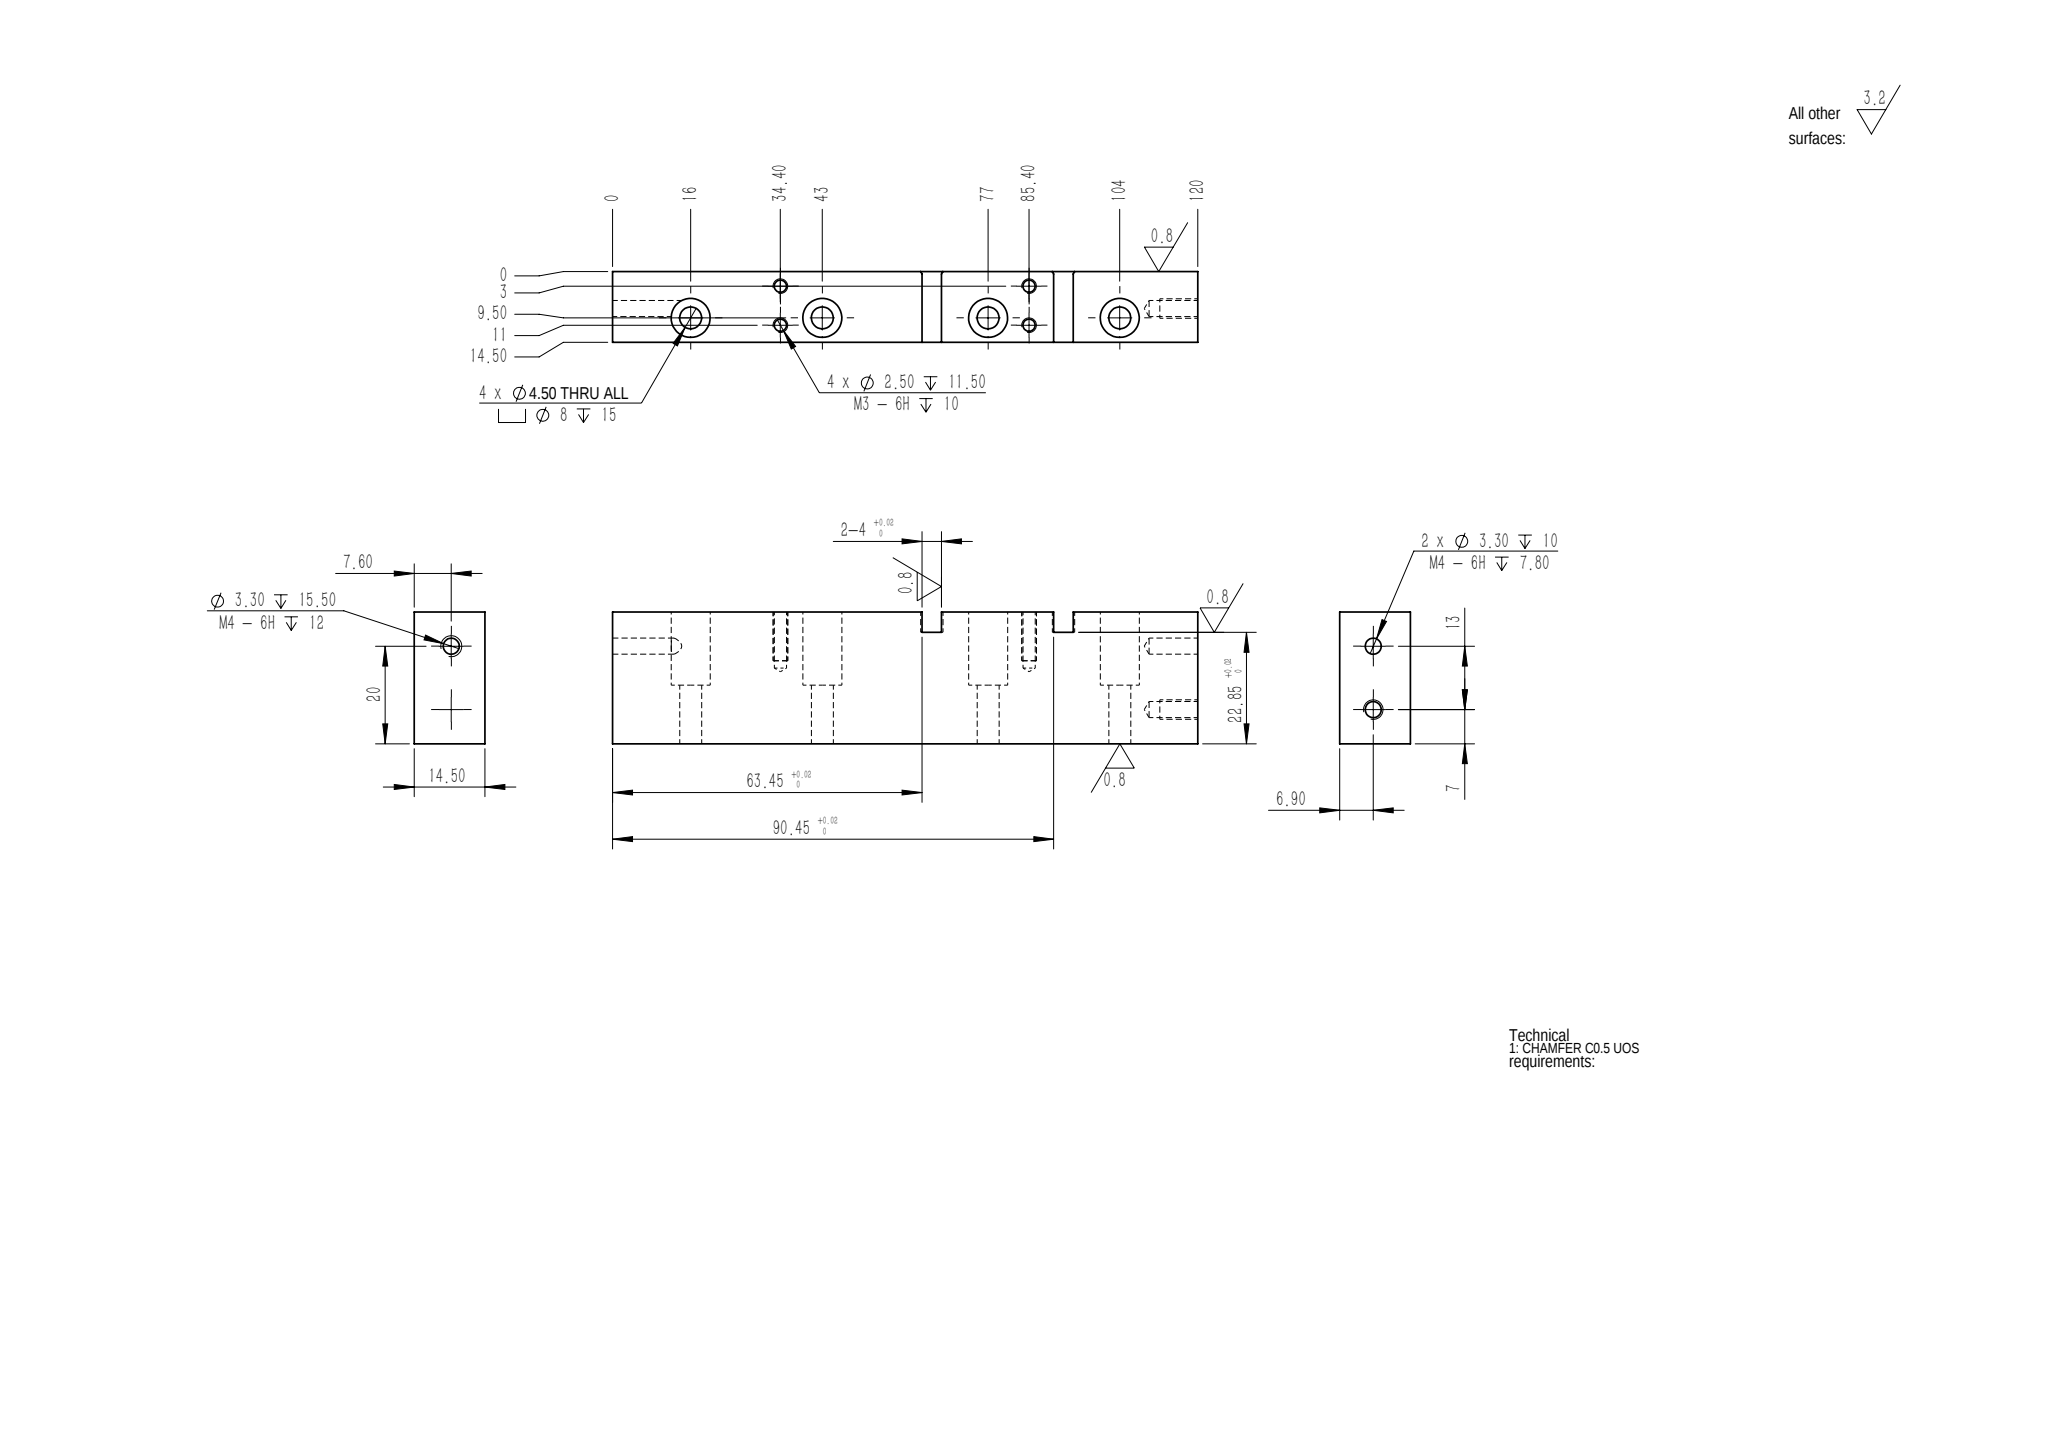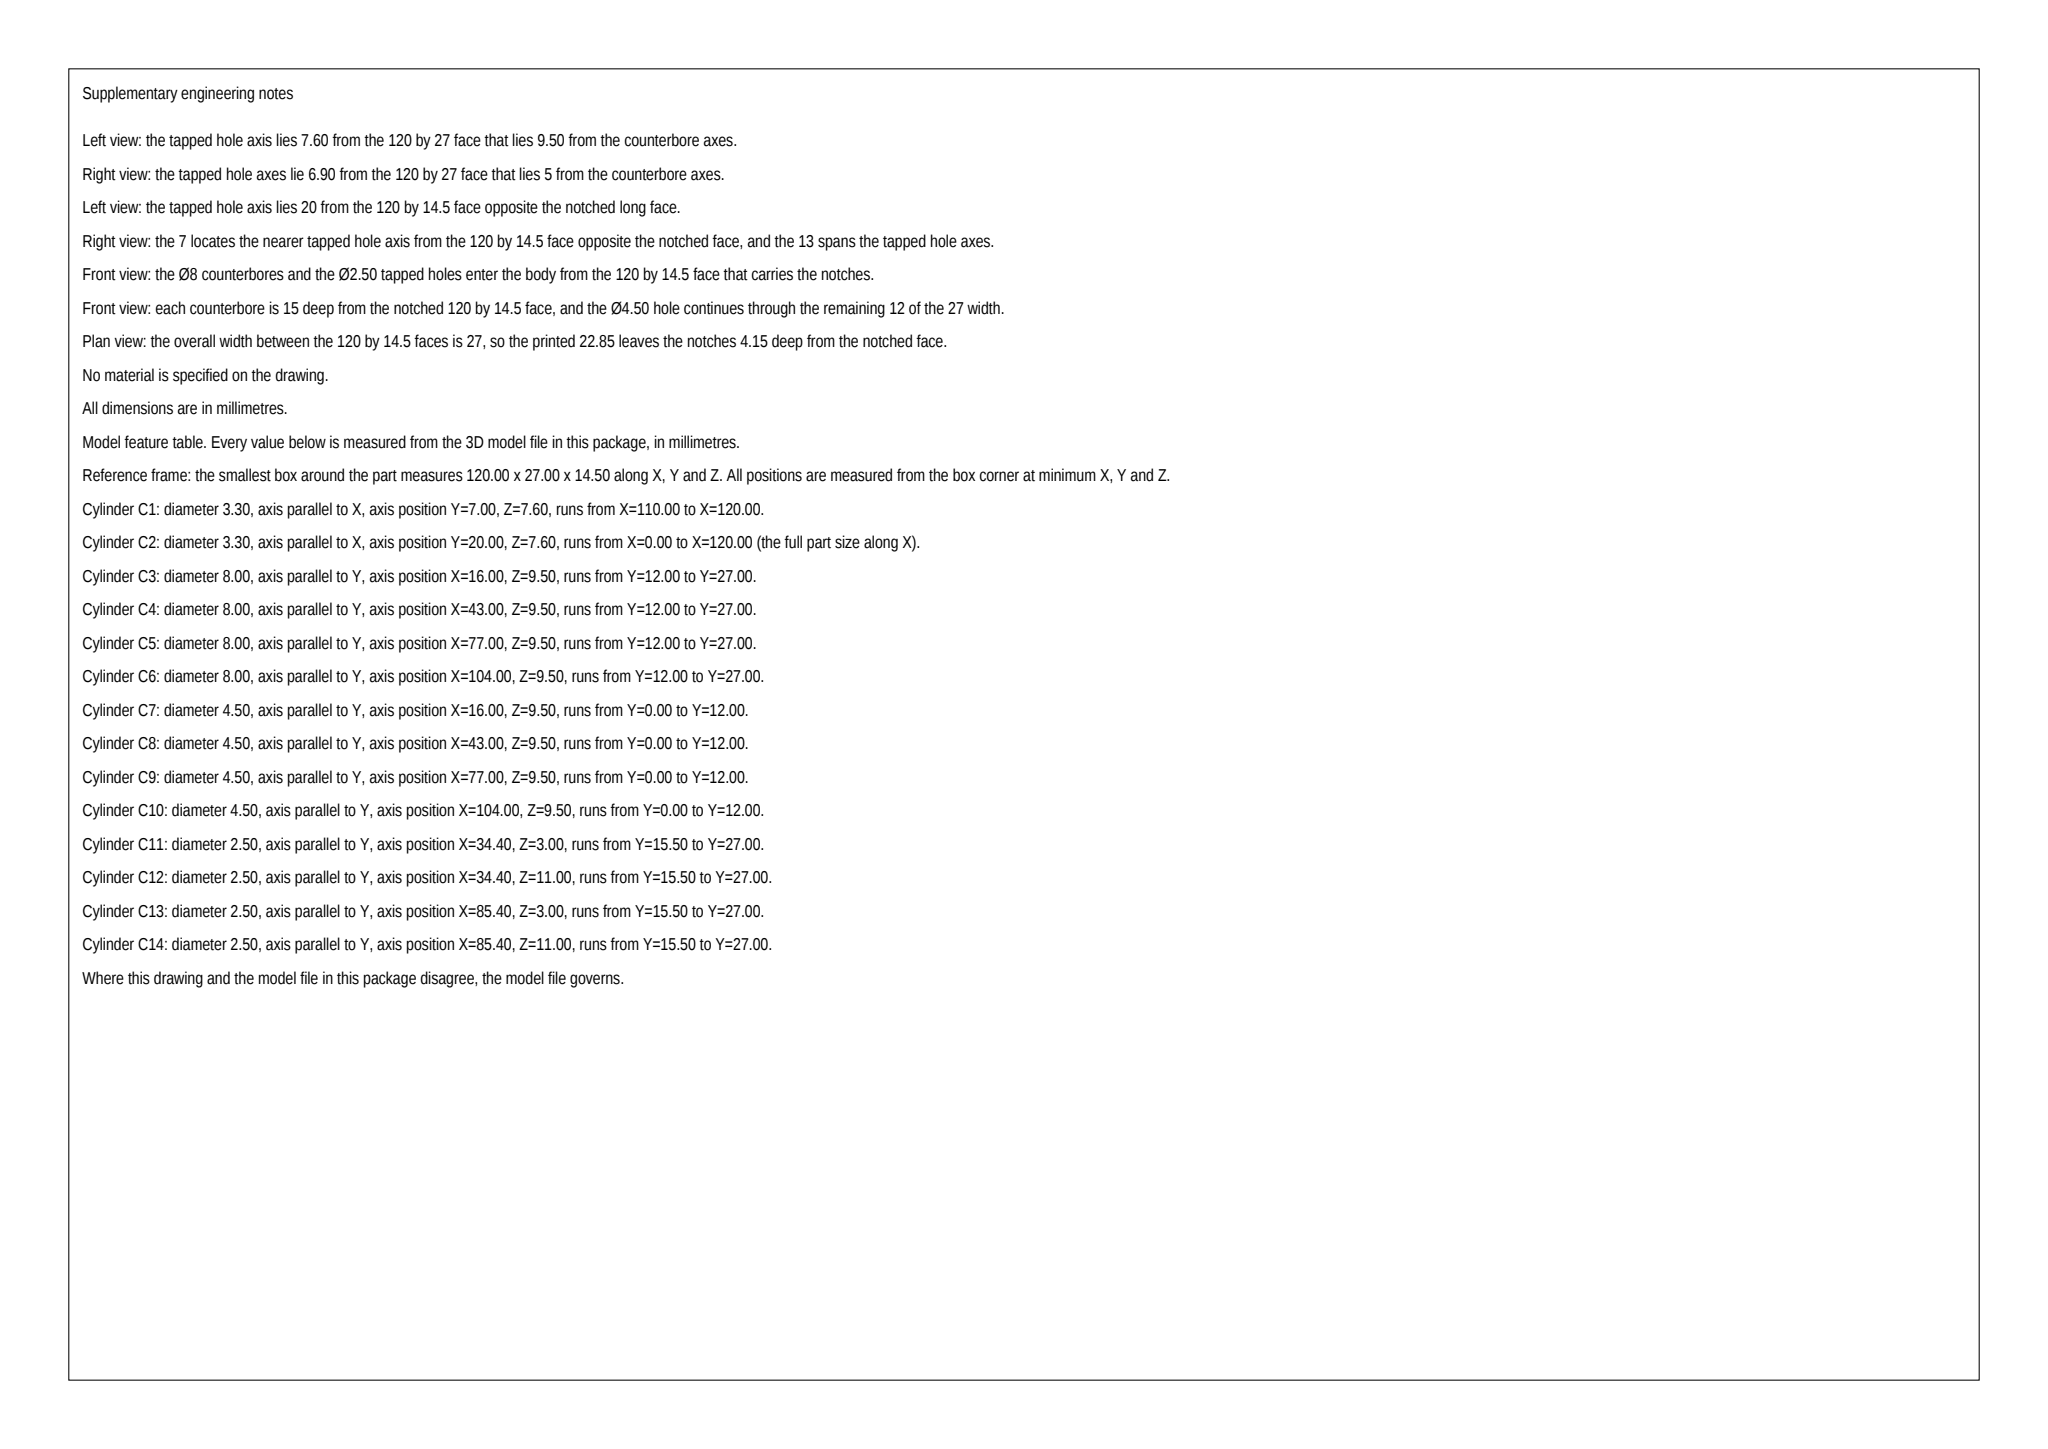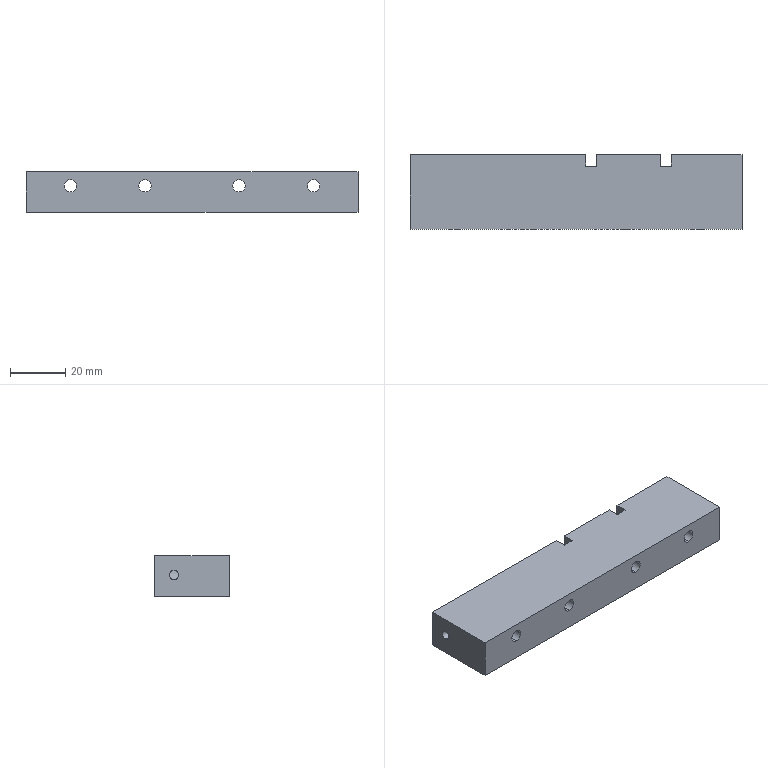Part | SolidWorks | mm | 1 solid | 64 faces | box 120 x 27 x 14.5 mm | volume 42203 mm3 | cylinder 30 | plane 22 | cone 12 | commonest cylinder face diameters 4.5 x8 8 x8 2.5 x8 3.3 x6
Drawing notes:
OVERALL WIDTH 27 (Y) - SEE END VIEWS | from the solid: bbox_xyz Y = 27.0; y-planes at 0.0 and 27.0
2-4 WIDE SLOTS DP 4.15 (27-22.85) FULL ACROSS TOP | from the solid: y-plane 22.85 vs 27.0 face; 2-4 +0.02/0 slots at x 63.45-67.45 and 90.45-94.45
build123d program:
from build123d import *
from OCP.BRepFilletAPI import BRepFilletAPI_MakeChamfer

# Parameters (mm, degrees)
SKETCH1_W                                       = 120
SKETCH1_H                                       = 27
BOSS_EXTRUDE1_DEPTH                             = 14.5
M4_TAPPED_HOLE2_D                               = 3.3
M4_TAPPED_HOLE2_DEPTH                           = 10
M4_TAPPED_HOLE2_TIP                             = 0.9914
M4_TAPPED_HOLE3_D                               = 3.3
M4_TAPPED_HOLE3_DEPTH                           = 15.5
M4_TAPPED_HOLE3_TIP                             = 0.9914
M3_TAPPED_HOLE1_D                               = 2.5
M3_TAPPED_HOLE1_DEPTH                           = 11.5
M3_TAPPED_HOLE1_TIP                             = 0.7511
M4_HEX_SOCKET_HEAD_CAP_SCREW_CBORE1_D           = 4.5
M4_HEX_SOCKET_HEAD_CAP_SCREW_CBORE1_CBORE_D     = 8
M4_HEX_SOCKET_HEAD_CAP_SCREW_CBORE1_CBORE_DEPTH = 15
SKETCH19_W                                      = 4
SKETCH19_H                                      = 14.5
CUT_EXTRUDE1_DEPTH                              = 4.15
CHAMFER1_SIZE                                   = 0.5
CHAMFER1_SIZE2                                  = 0.2887


with BuildPart() as part:
    # Sketch1 → Boss-Extrude1 (new body)
    with BuildSketch(Plane.XY):
        Rectangle(SKETCH1_W, SKETCH1_H)
    extrude(amount=BOSS_EXTRUDE1_DEPTH)

    # M4 Tapped Hole2
    with Locations(Plane(origin=(60, 0, 0), x_dir=(0, 0, 1), z_dir=(1, 0, 0))):
        with Locations((7.6, -6.5), (7.6, 6.5)):
            Hole(M4_TAPPED_HOLE2_D / 2, depth=M4_TAPPED_HOLE2_DEPTH)
            with Locations((0, 0, -(M4_TAPPED_HOLE2_DEPTH + M4_TAPPED_HOLE2_TIP / 2))):  # 118° drill point
                Cone(0, M4_TAPPED_HOLE2_D / 2, M4_TAPPED_HOLE2_TIP, mode=Mode.SUBTRACT)

    # M4 Tapped Hole3
    with Locations(Plane(origin=(-60, 0, 0), x_dir=(0, 0, -1), z_dir=(-1, 0, 0))):
        with Locations((-7.6, -6.5)):
            Hole(M4_TAPPED_HOLE3_D / 2, depth=M4_TAPPED_HOLE3_DEPTH)
            with Locations((0, 0, -(M4_TAPPED_HOLE3_DEPTH + M4_TAPPED_HOLE3_TIP / 2))):  # 118° drill point
                Cone(0, M4_TAPPED_HOLE3_D / 2, M4_TAPPED_HOLE3_TIP, mode=Mode.SUBTRACT)

    # M3 Tapped Hole1
    with Locations(Plane(origin=(0, 13.5, 0), x_dir=(1, 0, 0), z_dir=(0, 1, 0))):
        with Locations((-25.6, -3), (25.4, -3), (25.4, -11), (-25.6, -11)):
            Hole(M3_TAPPED_HOLE1_D / 2, depth=M3_TAPPED_HOLE1_DEPTH)
            with Locations((0, 0, -(M3_TAPPED_HOLE1_DEPTH + M3_TAPPED_HOLE1_TIP / 2))):  # 118° drill point
                Cone(0, M3_TAPPED_HOLE1_D / 2, M3_TAPPED_HOLE1_TIP, mode=Mode.SUBTRACT)

    # M4 Hex Socket Head Cap Screw CBORE1 (through all)
    with Locations(Plane(origin=(0, 13.5, 0), x_dir=(1, 0, 0), z_dir=(0, 1, 0))):
        with Locations((-44, -9.5), (-17, -9.5), (17, -9.5), (44, -9.5)):
            CounterBoreHole(M4_HEX_SOCKET_HEAD_CAP_SCREW_CBORE1_D / 2, M4_HEX_SOCKET_HEAD_CAP_SCREW_CBORE1_CBORE_D / 2, M4_HEX_SOCKET_HEAD_CAP_SCREW_CBORE1_CBORE_DEPTH)

    # Sketch19 → Cut-Extrude1 (cut)
    with BuildSketch(Plane(origin=(0, 13.5, 0), x_dir=(1, 0, 0), z_dir=(0, 1, 0))):
        with Locations((5.45, -7.25)):
            Rectangle(SKETCH19_W, SKETCH19_H)
        with Locations((32.45, -7.25)):
            Rectangle(SKETCH19_W, SKETCH19_H)
    extrude(amount=-CUT_EXTRUDE1_DEPTH, mode=Mode.SUBTRACT)

    # Chamfer1: one chamfer whose edges measure the first distance from different faces: ONE call of the kernel's chamfer builder (chamfer() names one face for all edges)
    chamfer1_edges_1 = [part.edges().sort_by_distance(p)[0] for p in [
        (3.45, 11.425, 0),
    ]]
    chamfer1_side_1 = [part.faces().sort_by_distance(p)[0] for p in [
        (3.45, 11.425, 7.25),
    ]]
    chamfer1_edges_2 = [part.edges().sort_by_distance(p)[0] for p in [
        (7.45, 11.425, 0),
    ]]
    chamfer1_side_2 = [part.faces().sort_by_distance(p)[0] for p in [
        (7.45, 11.425, 7.25),
    ]]
    chamfer1_edges_3 = [part.edges().sort_by_distance(p)[0] for p in [
        (34.45, 11.425, 0),
    ]]
    chamfer1_side_3 = [part.faces().sort_by_distance(p)[0] for p in [
        (34.45, 11.425, 7.25),
    ]]
    chamfer1_edges_4 = [part.edges().sort_by_distance(p)[0] for p in [
        (30.45, 11.425, 0),
    ]]
    chamfer1_side_4 = [part.faces().sort_by_distance(p)[0] for p in [
        (30.45, 11.425, 7.25),
    ]]
    chamfer1 = BRepFilletAPI_MakeChamfer(part.part.solid().wrapped)
    for e in chamfer1_edges_1:
        chamfer1.Add(CHAMFER1_SIZE, CHAMFER1_SIZE2, e.wrapped, chamfer1_side_1[0].wrapped)  # the first distance lies on this face
    for e in chamfer1_edges_2:
        chamfer1.Add(CHAMFER1_SIZE, CHAMFER1_SIZE2, e.wrapped, chamfer1_side_2[0].wrapped)  # the first distance lies on this face
    for e in chamfer1_edges_3:
        chamfer1.Add(CHAMFER1_SIZE, CHAMFER1_SIZE2, e.wrapped, chamfer1_side_3[0].wrapped)  # the first distance lies on this face
    for e in chamfer1_edges_4:
        chamfer1.Add(CHAMFER1_SIZE, CHAMFER1_SIZE2, e.wrapped, chamfer1_side_4[0].wrapped)  # the first distance lies on this face
    add(Compound.cast(chamfer1.Shape()), mode=Mode.REPLACE)


solid = part.part